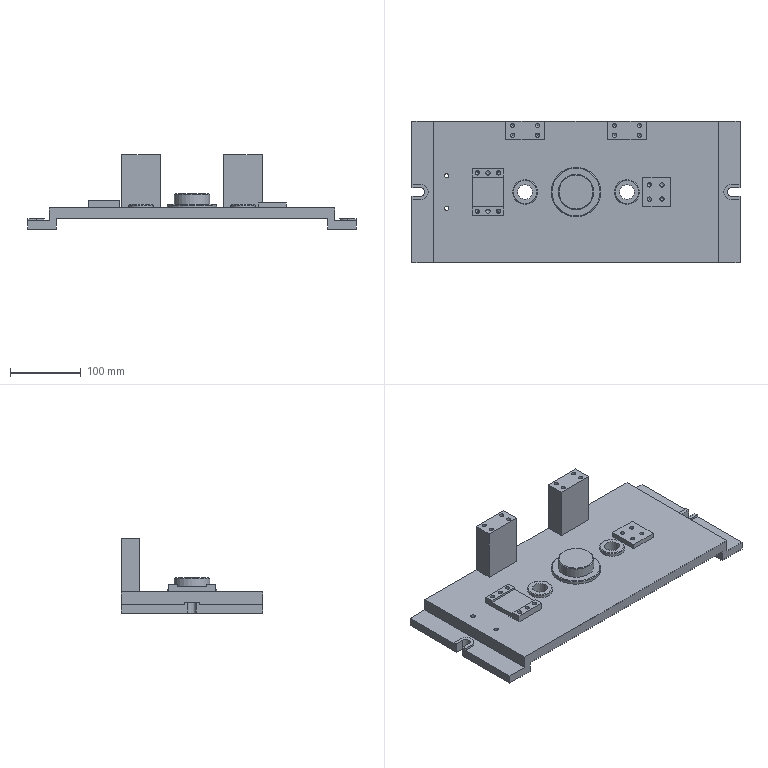Component | NX | JIG_BODY | 1 solid | 114 faces | volume 1700419 mm3 | plane 62 | cylinder 30 | cone 22 | commonest cylinder face diameters 6 x20 35 x2 21 x2 12 x2 22 x2 70 x1 50 x1